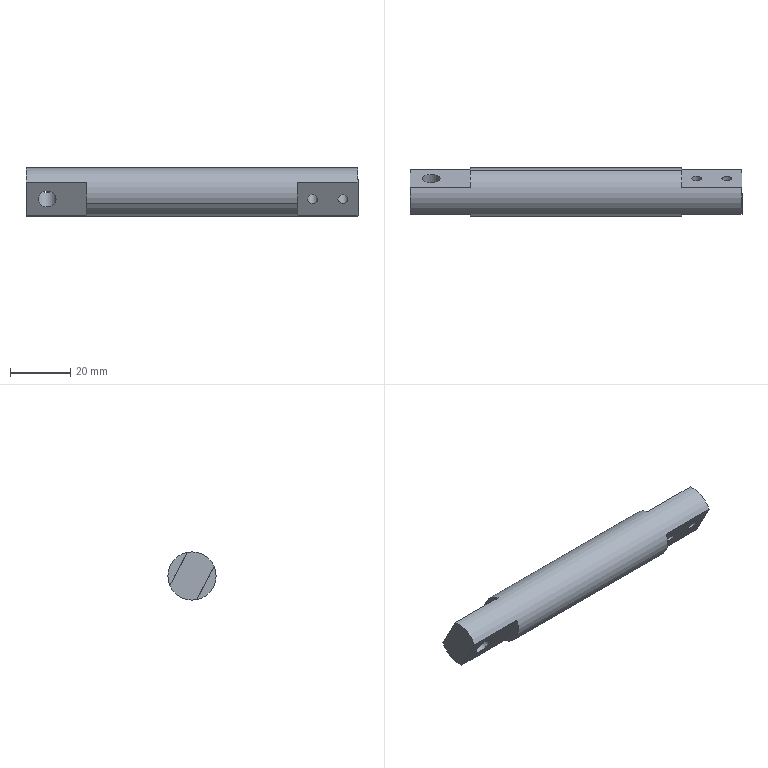Component | SolidWorks | BladeConnectingRod-1 | 1 solid | 18 faces | box 110 x 16 x 16 mm | volume 19575 mm3 | plane 10 | cylinder 8 | commonest cylinder face diameters 3.3 x4 6 x2 16 x2
build123d program:
from build123d import *

# Parameters (mm, degrees)
SKETCH1_R                    = 8
BOSS_EXTRUDE1_DEPTH          = 110
CUT_EXTRUDE1_DEPTH           = 20
F_6_0_6_DIAMETER_HOLE1_D     = 6
F_6_0_6_DIAMETER_HOLE1_DEPTH = 24
F_6_0_6_DIAMETER_HOLE1_TIP   = 1.803
CUT_EXTRUDE2_START           = -20
CUT_EXTRUDE2_DEPTH           = 20
M4_TAPPED_HOLE1_D            = 3.3
M4_TAPPED_HOLE1_DEPTH        = 13.5
M4_TAPPED_HOLE1_TIP          = 0.9914


with BuildPart() as part:
    # Sketch1 → Boss-Extrude1 (new body)
    with BuildSketch(Plane.XY):
        Circle(SKETCH1_R)
    extrude(amount=BOSS_EXTRUDE1_DEPTH)

    # Sketch2 → Cut-Extrude1 (cut)
    with BuildSketch(Plane(origin=(0, 0, 0), x_dir=(-1, 0, 0), z_dir=(0, 0, -1))):
        with BuildLine():
            Line((5, 6.245), (5, -6.245))
            ThreePointArc((5, -6.245), (8, 0), (5, 6.245))
        make_face()
        with BuildLine():
            Line((-5, 6.245), (-5, -6.245))
            ThreePointArc((-5, -6.245), (-8, 0), (-5, 6.245))
        make_face()
    extrude(amount=-CUT_EXTRUDE1_DEPTH, mode=Mode.SUBTRACT)

    # 6.0 _6_ Diameter Hole1
    with Locations(Plane(origin=(5, 0, 0), x_dir=(0, 0, -1), z_dir=(1, 0, 0))):
        with Locations((-7, 0)):
            Hole(F_6_0_6_DIAMETER_HOLE1_D / 2, depth=F_6_0_6_DIAMETER_HOLE1_DEPTH)
            with Locations((0, 0, -(F_6_0_6_DIAMETER_HOLE1_DEPTH + F_6_0_6_DIAMETER_HOLE1_TIP / 2))):  # 118° drill point
                Cone(0, F_6_0_6_DIAMETER_HOLE1_D / 2, F_6_0_6_DIAMETER_HOLE1_TIP, mode=Mode.SUBTRACT)

    # Sketch5 → Cut-Extrude2 (cut)
    with BuildSketch(Plane.XY.offset(110).offset(CUT_EXTRUDE2_START)):
        with BuildLine():
            Line((-5, 6.245), (-5, -6.245))
            ThreePointArc((-5, -6.245), (-8, 0), (-5, 6.245))
        make_face()
        with BuildLine():
            Line((5, 6.245), (5, -6.245))
            ThreePointArc((5, -6.245), (8, 0), (5, 6.245))
        make_face()
    extrude(amount=CUT_EXTRUDE2_DEPTH, mode=Mode.SUBTRACT)

    # M4 Tapped Hole1
    with Locations(Plane(origin=(5, 0, 0), x_dir=(0, 0, -1), z_dir=(1, 0, 0))):
        with Locations((-105, 0), (-95, 0)):
            Hole(M4_TAPPED_HOLE1_D / 2, depth=M4_TAPPED_HOLE1_DEPTH)
            with Locations((0, 0, -(M4_TAPPED_HOLE1_DEPTH + M4_TAPPED_HOLE1_TIP / 2))):  # 118° drill point
                Cone(0, M4_TAPPED_HOLE1_D / 2, M4_TAPPED_HOLE1_TIP, mode=Mode.SUBTRACT)


solid = part.part

# Placed as in the assembly
solid = solid.moved(Location((-280.317, -22.413, 172.524), (117.698, 90, 0)))
STEP:
#1=CARTESIAN_POINT('',(-6.837,-0.7081,6.884));
#2=VERTEX_POINT('',#1);
#3=CARTESIAN_POINT('',(-6.967,-0.7081,6.884));
#4=VERTEX_POINT('',#3);
#5=CARTESIAN_POINT('',(-6.902,-0.7081,6.884));
#6=DIRECTION('',(0.,-0.8854,-0.4648));
#7=DIRECTION('',(-1.,-0.,0.));
#8=AXIS2_PLACEMENT_3D('',#5,#6,#7);
#9=CIRCLE('',#8,0.06496);
#10=EDGE_CURVE('',#2,#4,#9,.T.);
#11=ORIENTED_EDGE('',*,*,#10,.F.);
#12=CARTESIAN_POINT('',(-6.837,-1.057,6.701));
#13=VERTEX_POINT('',#12);
#14=CARTESIAN_POINT('',(-6.837,-1.057,6.701));
#15=DIRECTION('',(0.,-0.8854,-0.4648));
#16=VECTOR('',#15,39.37);
#17=LINE('',#14,#16);
#18=EDGE_CURVE('',#2,#13,#17,.T.);
#19=ORIENTED_EDGE('',*,*,#18,.T.);
#20=CARTESIAN_POINT('',(-6.967,-1.057,6.701));
#21=VERTEX_POINT('',#20);
#22=CARTESIAN_POINT('',(-6.902,-1.057,6.701));
#23=DIRECTION('',(0.,-0.8854,-0.4648));
#24=DIRECTION('',(-1.,-0.,0.));
#25=AXIS2_PLACEMENT_3D('',#22,#23,#24);
#26=CIRCLE('',#25,0.06496);
#27=EDGE_CURVE('',#13,#21,#26,.T.);
#28=ORIENTED_EDGE('',*,*,#27,.T.);
#29=CARTESIAN_POINT('',(-6.967,-1.057,6.701));
#30=DIRECTION('',(0.,-0.8854,-0.4648));
#31=VECTOR('',#30,39.37);
#32=LINE('',#29,#31);
#33=EDGE_CURVE('',#4,#21,#32,.T.);
#34=ORIENTED_EDGE('',*,*,#33,.F.);
#35=EDGE_LOOP('',(#11,#19,#28,#34));
#36=FACE_OUTER_BOUND('',#35,.T.);
#37=CARTESIAN_POINT('',(-6.902,-1.057,6.701));
#38=DIRECTION('',(0.,-0.8854,-0.4648));
#39=DIRECTION('',(-1.,-0.,0.));
#40=AXIS2_PLACEMENT_3D('',#37,#38,#39);
#41=CYLINDRICAL_SURFACE('',#40,0.06496);
#42=ADVANCED_FACE('',(#36),#41,.F.);
#43=CARTESIAN_POINT('',(-7.231,-0.7081,6.884));
#44=VERTEX_POINT('',#43);
#45=CARTESIAN_POINT('',(-7.361,-0.7081,6.884));
#46=VERTEX_POINT('',#45);
#47=CARTESIAN_POINT('',(-7.296,-0.7081,6.884));
#48=DIRECTION('',(0.,-0.8854,-0.4648));
#49=DIRECTION('',(-1.,-0.,0.));
#50=AXIS2_PLACEMENT_3D('',#47,#48,#49);
#51=CIRCLE('',#50,0.06496);
#52=EDGE_CURVE('',#44,#46,#51,.T.);
#53=ORIENTED_EDGE('',*,*,#52,.F.);
#54=CARTESIAN_POINT('',(-7.231,-1.057,6.701));
#55=VERTEX_POINT('',#54);
#56=CARTESIAN_POINT('',(-7.231,-1.057,6.701));
#57=DIRECTION('',(0.,-0.8854,-0.4648));
#58=VECTOR('',#57,39.37);
#59=LINE('',#56,#58);
#60=EDGE_CURVE('',#44,#55,#59,.T.);
#61=ORIENTED_EDGE('',*,*,#60,.T.);
#62=CARTESIAN_POINT('',(-7.361,-1.057,6.701));
#63=VERTEX_POINT('',#62);
#64=CARTESIAN_POINT('',(-7.296,-1.057,6.701));
#65=DIRECTION('',(0.,-0.8854,-0.4648));
#66=DIRECTION('',(-1.,-0.,0.));
#67=AXIS2_PLACEMENT_3D('',#64,#65,#66);
#68=CIRCLE('',#67,0.06496);
#69=EDGE_CURVE('',#55,#63,#68,.T.);
#70=ORIENTED_EDGE('',*,*,#69,.T.);
#71=CARTESIAN_POINT('',(-7.361,-1.057,6.701));
#72=DIRECTION('',(0.,-0.8854,-0.4648));
#73=VECTOR('',#72,39.37);
#74=LINE('',#71,#73);
#75=EDGE_CURVE('',#46,#63,#74,.T.);
#76=ORIENTED_EDGE('',*,*,#75,.F.);
#77=EDGE_LOOP('',(#53,#61,#70,#76));
#78=FACE_OUTER_BOUND('',#77,.T.);
#79=CARTESIAN_POINT('',(-7.296,-1.057,6.701));
#80=DIRECTION('',(0.,-0.8854,-0.4648));
#81=DIRECTION('',(-1.,-0.,0.));
#82=AXIS2_PLACEMENT_3D('',#79,#80,#81);
#83=CYLINDRICAL_SURFACE('',#82,0.06496);
#84=ADVANCED_FACE('',(#78),#83,.F.);
#85=CARTESIAN_POINT('',(-10.642,-0.7081,6.884));
#86=VERTEX_POINT('',#85);
#87=CARTESIAN_POINT('',(-10.879,-0.7081,6.884));
#88=VERTEX_POINT('',#87);
#89=CARTESIAN_POINT('',(-10.76,-0.7081,6.884));
#90=DIRECTION('',(0.,-0.8854,-0.4648));
#91=DIRECTION('',(-1.,-0.,0.));
#92=AXIS2_PLACEMENT_3D('',#89,#90,#91);
#93=CIRCLE('',#92,0.1181);
#94=EDGE_CURVE('',#86,#88,#93,.T.);
#95=ORIENTED_EDGE('',*,*,#94,.F.);
#96=CARTESIAN_POINT('',(-10.642,-1.057,6.701));
#97=VERTEX_POINT('',#96);
#98=CARTESIAN_POINT('',(-10.642,-1.057,6.701));
#99=DIRECTION('',(0.,-0.8854,-0.4648));
#100=VECTOR('',#99,39.37);
#101=LINE('',#98,#100);
#102=EDGE_CURVE('',#86,#97,#101,.T.);
#103=ORIENTED_EDGE('',*,*,#102,.T.);
#104=CARTESIAN_POINT('',(-10.879,-1.057,6.701));
#105=VERTEX_POINT('',#104);
#106=CARTESIAN_POINT('',(-10.76,-1.057,6.701));
#107=DIRECTION('',(0.,-0.8854,-0.4648));
#108=DIRECTION('',(-1.,-0.,0.));
#109=AXIS2_PLACEMENT_3D('',#106,#107,#108);
#110=CIRCLE('',#109,0.1181);
#111=EDGE_CURVE('',#97,#105,#110,.T.);
#112=ORIENTED_EDGE('',*,*,#111,.T.);
#113=CARTESIAN_POINT('',(-10.879,-1.057,6.701));
#114=DIRECTION('',(0.,-0.8854,-0.4648));
#115=VECTOR('',#114,39.37);
#116=LINE('',#113,#115);
#117=EDGE_CURVE('',#88,#105,#116,.T.);
#118=ORIENTED_EDGE('',*,*,#117,.F.);
#119=EDGE_LOOP('',(#95,#103,#112,#118));
#120=FACE_OUTER_BOUND('',#119,.T.);
#121=CARTESIAN_POINT('',(-10.76,-1.057,6.701));
#122=DIRECTION('',(0.,-0.8854,-0.4648));
#123=DIRECTION('',(-1.,-0.,0.));
#124=AXIS2_PLACEMENT_3D('',#121,#122,#123);
#125=CYLINDRICAL_SURFACE('',#124,0.1181);
#126=ADVANCED_FACE('',(#120),#125,.F.);
#127=CARTESIAN_POINT('',(-7.493,-1.161,6.646));
#128=VERTEX_POINT('',#127);
#129=CARTESIAN_POINT('',(-7.493,-0.9424,6.483));
#130=VERTEX_POINT('',#129);
#131=CARTESIAN_POINT('',(-7.493,-0.8824,6.792));
#132=DIRECTION('',(1.,0.,0.));
#133=DIRECTION('',(0.,-0.8854,-0.4648));
#134=AXIS2_PLACEMENT_3D('',#131,#132,#133);
#135=CIRCLE('',#134,0.315);
#136=EDGE_CURVE('',#128,#130,#135,.T.);
#137=ORIENTED_EDGE('',*,*,#136,.F.);
#138=CARTESIAN_POINT('',(-10.249,-1.161,6.646));
#139=VERTEX_POINT('',#138);
#140=CARTESIAN_POINT('',(-6.705,-1.161,6.646));
#141=DIRECTION('',(-1.,-0.,-0.));
#142=VECTOR('',#141,39.37);
#143=LINE('',#140,#142);
#144=EDGE_CURVE('',#128,#139,#143,.T.);
#145=ORIENTED_EDGE('',*,*,#144,.T.);
#146=CARTESIAN_POINT('',(-10.249,-0.9424,6.483));
#147=VERTEX_POINT('',#146);
#148=CARTESIAN_POINT('',(-10.249,-0.8824,6.792));
#149=DIRECTION('',(-1.,-0.,-0.));
#150=DIRECTION('',(0.,0.8854,0.4648));
#151=AXIS2_PLACEMENT_3D('',#148,#149,#150);
#152=CIRCLE('',#151,0.315);
#153=EDGE_CURVE('',#147,#139,#152,.T.);
#154=ORIENTED_EDGE('',*,*,#153,.F.);
#155=CARTESIAN_POINT('',(-11.036,-0.9424,6.483));
#156=VERTEX_POINT('',#155);
#157=CARTESIAN_POINT('',(-10.249,-0.9424,6.483));
#158=DIRECTION('',(-1.,-0.,-0.));
#159=VECTOR('',#158,39.37);
#160=LINE('',#157,#159);
#161=EDGE_CURVE('',#147,#156,#160,.T.);
#162=ORIENTED_EDGE('',*,*,#161,.T.);
#163=CARTESIAN_POINT('',(-11.036,-0.5938,6.666));
#164=VERTEX_POINT('',#163);
#165=CARTESIAN_POINT('',(-11.036,-0.8824,6.792));
#166=DIRECTION('',(1.,0.,0.));
#167=DIRECTION('',(0.,-0.8854,-0.4648));
#168=AXIS2_PLACEMENT_3D('',#165,#166,#167);
#169=CIRCLE('',#168,0.315);
#170=EDGE_CURVE('',#156,#164,#169,.T.);
#171=ORIENTED_EDGE('',*,*,#170,.T.);
#172=CARTESIAN_POINT('',(-10.249,-0.5938,6.666));
#173=VERTEX_POINT('',#172);
#174=CARTESIAN_POINT('',(-10.249,-0.5938,6.666));
#175=DIRECTION('',(-1.,-0.,-0.));
#176=VECTOR('',#175,39.37);
#177=LINE('',#174,#176);
#178=EDGE_CURVE('',#173,#164,#177,.T.);
#179=ORIENTED_EDGE('',*,*,#178,.F.);
#180=CARTESIAN_POINT('',(-10.249,-0.6035,6.939));
#181=VERTEX_POINT('',#180);
#182=CARTESIAN_POINT('',(-10.249,-0.8824,6.792));
#183=DIRECTION('',(-1.,-0.,-0.));
#184=DIRECTION('',(0.,0.8854,0.4648));
#185=AXIS2_PLACEMENT_3D('',#182,#183,#184);
#186=CIRCLE('',#185,0.315);
#187=EDGE_CURVE('',#181,#173,#186,.T.);
#188=ORIENTED_EDGE('',*,*,#187,.F.);
#189=CARTESIAN_POINT('',(-7.493,-0.6035,6.939));
#190=VERTEX_POINT('',#189);
#191=CARTESIAN_POINT('',(-6.705,-0.6035,6.939));
#192=DIRECTION('',(-1.,-0.,-0.));
#193=VECTOR('',#192,39.37);
#194=LINE('',#191,#193);
#195=EDGE_CURVE('',#190,#181,#194,.T.);
#196=ORIENTED_EDGE('',*,*,#195,.F.);
#197=CARTESIAN_POINT('',(-7.493,-0.5938,6.666));
#198=VERTEX_POINT('',#197);
#199=CARTESIAN_POINT('',(-7.493,-0.8824,6.792));
#200=DIRECTION('',(1.,0.,0.));
#201=DIRECTION('',(0.,-0.8854,-0.4648));
#202=AXIS2_PLACEMENT_3D('',#199,#200,#201);
#203=CIRCLE('',#202,0.315);
#204=EDGE_CURVE('',#198,#190,#203,.T.);
#205=ORIENTED_EDGE('',*,*,#204,.F.);
#206=CARTESIAN_POINT('',(-6.705,-0.5938,6.666));
#207=VERTEX_POINT('',#206);
#208=CARTESIAN_POINT('',(-7.493,-0.5938,6.666));
#209=DIRECTION('',(1.,0.,0.));
#210=VECTOR('',#209,39.37);
#211=LINE('',#208,#210);
#212=EDGE_CURVE('',#198,#207,#211,.T.);
#213=ORIENTED_EDGE('',*,*,#212,.T.);
#214=CARTESIAN_POINT('',(-6.705,-0.9424,6.483));
#215=VERTEX_POINT('',#214);
#216=CARTESIAN_POINT('',(-6.705,-0.8824,6.792));
#217=DIRECTION('',(1.,0.,0.));
#218=DIRECTION('',(0.,-0.8854,-0.4648));
#219=AXIS2_PLACEMENT_3D('',#216,#217,#218);
#220=CIRCLE('',#219,0.315);
#221=EDGE_CURVE('',#215,#207,#220,.T.);
#222=ORIENTED_EDGE('',*,*,#221,.F.);
#223=CARTESIAN_POINT('',(-7.493,-0.9424,6.483));
#224=DIRECTION('',(1.,0.,0.));
#225=VECTOR('',#224,39.37);
#226=LINE('',#223,#225);
#227=EDGE_CURVE('',#130,#215,#226,.T.);
#228=ORIENTED_EDGE('',*,*,#227,.F.);
#229=EDGE_LOOP('',(#137,#145,#154,#162,#171,#179,#188,#196,#205,#213,#222,#228));
#230=FACE_OUTER_BOUND('',#229,.T.);
#231=CARTESIAN_POINT('',(-6.705,-0.8824,6.792));
#232=DIRECTION('',(-1.,-0.,-0.));
#233=DIRECTION('',(-0.,0.8854,0.4648));
#234=AXIS2_PLACEMENT_3D('',#231,#232,#233);
#235=CYLINDRICAL_SURFACE('',#234,0.315);
#236=ADVANCED_FACE('',(#230),#235,.T.);
#237=ORIENTED_EDGE('',*,*,#144,.F.);
#238=CARTESIAN_POINT('',(-7.493,-1.171,6.918));
#239=VERTEX_POINT('',#238);
#240=CARTESIAN_POINT('',(-7.493,-0.8824,6.792));
#241=DIRECTION('',(1.,0.,0.));
#242=DIRECTION('',(0.,-0.8854,-0.4648));
#243=AXIS2_PLACEMENT_3D('',#240,#241,#242);
#244=CIRCLE('',#243,0.315);
#245=EDGE_CURVE('',#239,#128,#244,.T.);
#246=ORIENTED_EDGE('',*,*,#245,.F.);
#247=CARTESIAN_POINT('',(-6.705,-1.171,6.918));
#248=VERTEX_POINT('',#247);
#249=CARTESIAN_POINT('',(-7.493,-1.171,6.918));
#250=DIRECTION('',(1.,0.,0.));
#251=VECTOR('',#250,39.37);
#252=LINE('',#249,#251);
#253=EDGE_CURVE('',#239,#248,#252,.T.);
#254=ORIENTED_EDGE('',*,*,#253,.T.);
#255=CARTESIAN_POINT('',(-6.705,-0.8224,7.101));
#256=VERTEX_POINT('',#255);
#257=CARTESIAN_POINT('',(-6.705,-0.8824,6.792));
#258=DIRECTION('',(1.,0.,0.));
#259=DIRECTION('',(0.,-0.8854,-0.4648));
#260=AXIS2_PLACEMENT_3D('',#257,#258,#259);
#261=CIRCLE('',#260,0.315);
#262=EDGE_CURVE('',#256,#248,#261,.T.);
#263=ORIENTED_EDGE('',*,*,#262,.F.);
#264=CARTESIAN_POINT('',(-7.493,-0.8224,7.101));
#265=VERTEX_POINT('',#264);
#266=CARTESIAN_POINT('',(-7.493,-0.8224,7.101));
#267=DIRECTION('',(1.,0.,0.));
#268=VECTOR('',#267,39.37);
#269=LINE('',#266,#268);
#270=EDGE_CURVE('',#265,#256,#269,.T.);
#271=ORIENTED_EDGE('',*,*,#270,.F.);
#272=CARTESIAN_POINT('',(-7.493,-0.8824,6.792));
#273=DIRECTION('',(1.,0.,0.));
#274=DIRECTION('',(0.,-0.8854,-0.4648));
#275=AXIS2_PLACEMENT_3D('',#272,#273,#274);
#276=CIRCLE('',#275,0.315);
#277=EDGE_CURVE('',#190,#265,#276,.T.);
#278=ORIENTED_EDGE('',*,*,#277,.F.);
#279=ORIENTED_EDGE('',*,*,#195,.T.);
#280=CARTESIAN_POINT('',(-10.249,-0.8224,7.101));
#281=VERTEX_POINT('',#280);
#282=CARTESIAN_POINT('',(-10.249,-0.8824,6.792));
#283=DIRECTION('',(-1.,-0.,-0.));
#284=DIRECTION('',(0.,0.8854,0.4648));
#285=AXIS2_PLACEMENT_3D('',#282,#283,#284);
#286=CIRCLE('',#285,0.315);
#287=EDGE_CURVE('',#281,#181,#286,.T.);
#288=ORIENTED_EDGE('',*,*,#287,.F.);
#289=CARTESIAN_POINT('',(-11.036,-0.8224,7.101));
#290=VERTEX_POINT('',#289);
#291=CARTESIAN_POINT('',(-10.249,-0.8224,7.101));
#292=DIRECTION('',(-1.,-0.,-0.));
#293=VECTOR('',#292,39.37);
#294=LINE('',#291,#293);
#295=EDGE_CURVE('',#281,#290,#294,.T.);
#296=ORIENTED_EDGE('',*,*,#295,.T.);
#297=CARTESIAN_POINT('',(-11.036,-1.171,6.918));
#298=VERTEX_POINT('',#297);
#299=CARTESIAN_POINT('',(-11.036,-0.8824,6.792));
#300=DIRECTION('',(1.,0.,0.));
#301=DIRECTION('',(0.,-0.8854,-0.4648));
#302=AXIS2_PLACEMENT_3D('',#299,#300,#301);
#303=CIRCLE('',#302,0.315);
#304=EDGE_CURVE('',#290,#298,#303,.T.);
#305=ORIENTED_EDGE('',*,*,#304,.T.);
#306=CARTESIAN_POINT('',(-10.249,-1.171,6.918));
#307=VERTEX_POINT('',#306);
#308=CARTESIAN_POINT('',(-10.249,-1.171,6.918));
#309=DIRECTION('',(-1.,-0.,-0.));
#310=VECTOR('',#309,39.37);
#311=LINE('',#308,#310);
#312=EDGE_CURVE('',#307,#298,#311,.T.);
#313=ORIENTED_EDGE('',*,*,#312,.F.);
#314=CARTESIAN_POINT('',(-10.249,-0.8824,6.792));
#315=DIRECTION('',(-1.,-0.,-0.));
#316=DIRECTION('',(0.,0.8854,0.4648));
#317=AXIS2_PLACEMENT_3D('',#314,#315,#316);
#318=CIRCLE('',#317,0.315);
#319=EDGE_CURVE('',#139,#307,#318,.T.);
#320=ORIENTED_EDGE('',*,*,#319,.F.);
#321=EDGE_LOOP('',(#237,#246,#254,#263,#271,#278,#279,#288,#296,#305,#313,#320));
#322=FACE_OUTER_BOUND('',#321,.T.);
#323=CARTESIAN_POINT('',(-6.705,-0.8824,6.792));
#324=DIRECTION('',(-1.,-0.,-0.));
#325=DIRECTION('',(-0.,0.8854,0.4648));
#326=AXIS2_PLACEMENT_3D('',#323,#324,#325);
#327=CYLINDRICAL_SURFACE('',#326,0.315);
#328=ADVANCED_FACE('',(#322),#327,.T.);
#329=CARTESIAN_POINT('',(-6.705,-0.5938,6.666));
#330=DIRECTION('',(-0.,0.4648,-0.8854));
#331=VECTOR('',#330,39.37);
#332=LINE('',#329,#331);
#333=EDGE_CURVE('',#256,#207,#332,.T.);
#334=ORIENTED_EDGE('',*,*,#333,.F.);
#335=ORIENTED_EDGE('',*,*,#262,.T.);
#336=CARTESIAN_POINT('',(-6.705,-0.9424,6.483));
#337=DIRECTION('',(0.,-0.4648,0.8854));
#338=VECTOR('',#337,39.37);
#339=LINE('',#336,#338);
#340=EDGE_CURVE('',#215,#248,#339,.T.);
#341=ORIENTED_EDGE('',*,*,#340,.F.);
#342=ORIENTED_EDGE('',*,*,#221,.T.);
#343=EDGE_LOOP('',(#334,#335,#341,#342));
#344=FACE_OUTER_BOUND('',#343,.T.);
#345=CARTESIAN_POINT('',(-6.705,-0.8824,6.792));
#346=DIRECTION('',(1.,0.,0.));
#347=DIRECTION('',(0.,-0.8854,-0.4648));
#348=AXIS2_PLACEMENT_3D('',#345,#346,#347);
#349=PLANE('',#348);
#350=ADVANCED_FACE('',(#344),#349,.T.);
#351=ORIENTED_EDGE('',*,*,#304,.F.);
#352=CARTESIAN_POINT('',(-11.036,-0.5938,6.666));
#353=DIRECTION('',(0.,-0.4648,0.8854));
#354=VECTOR('',#353,39.37);
#355=LINE('',#352,#354);
#356=EDGE_CURVE('',#164,#290,#355,.T.);
#357=ORIENTED_EDGE('',*,*,#356,.F.);
#358=ORIENTED_EDGE('',*,*,#170,.F.);
#359=CARTESIAN_POINT('',(-11.036,-0.9424,6.483));
#360=DIRECTION('',(-0.,0.4648,-0.8854));
#361=VECTOR('',#360,39.37);
#362=LINE('',#359,#361);
#363=EDGE_CURVE('',#298,#156,#362,.T.);
#364=ORIENTED_EDGE('',*,*,#363,.F.);
#365=EDGE_LOOP('',(#351,#357,#358,#364));
#366=FACE_OUTER_BOUND('',#365,.T.);
#367=CARTESIAN_POINT('',(-11.036,-0.8824,6.792));
#368=DIRECTION('',(1.,0.,0.));
#369=DIRECTION('',(0.,-0.8854,-0.4648));
#370=AXIS2_PLACEMENT_3D('',#367,#368,#369);
#371=PLANE('',#370);
#372=ADVANCED_FACE('',(#366),#371,.F.);
#373=CARTESIAN_POINT('',(-10.76,-1.057,6.701));
#374=DIRECTION('',(0.,-0.8854,-0.4648));
#375=DIRECTION('',(-1.,-0.,0.));
#376=AXIS2_PLACEMENT_3D('',#373,#374,#375);
#377=CIRCLE('',#376,0.1181);
#378=EDGE_CURVE('',#105,#97,#377,.T.);
#379=ORIENTED_EDGE('',*,*,#378,.F.);
#380=ORIENTED_EDGE('',*,*,#111,.F.);
#381=EDGE_LOOP('',(#379,#380));
#382=FACE_BOUND('',#381,.T.);
#383=ORIENTED_EDGE('',*,*,#363,.T.);
#384=ORIENTED_EDGE('',*,*,#161,.F.);
#385=CARTESIAN_POINT('',(-10.249,-0.9424,6.483));
#386=DIRECTION('',(-0.,0.4648,-0.8854));
#387=VECTOR('',#386,39.37);
#388=LINE('',#385,#387);
#389=EDGE_CURVE('',#307,#147,#388,.T.);
#390=ORIENTED_EDGE('',*,*,#389,.F.);
#391=ORIENTED_EDGE('',*,*,#312,.T.);
#392=EDGE_LOOP('',(#383,#384,#390,#391));
#393=FACE_OUTER_BOUND('',#392,.T.);
#394=CARTESIAN_POINT('',(-10.249,-0.9424,6.483));
#395=DIRECTION('',(-0.,0.8854,0.4648));
#396=DIRECTION('',(1.,0.,0.));
#397=AXIS2_PLACEMENT_3D('',#394,#395,#396);
#398=PLANE('',#397);
#399=ADVANCED_FACE('',(#382,#393),#398,.F.);
#400=ORIENTED_EDGE('',*,*,#153,.T.);
#401=ORIENTED_EDGE('',*,*,#319,.T.);
#402=ORIENTED_EDGE('',*,*,#389,.T.);
#403=EDGE_LOOP('',(#400,#401,#402));
#404=FACE_OUTER_BOUND('',#403,.T.);
#405=CARTESIAN_POINT('',(-10.249,-0.8824,6.792));
#406=DIRECTION('',(-1.,-0.,-0.));
#407=DIRECTION('',(-0.,0.8854,0.4648));
#408=AXIS2_PLACEMENT_3D('',#405,#406,#407);
#409=PLANE('',#408);
#410=ADVANCED_FACE('',(#404),#409,.T.);
#411=CARTESIAN_POINT('',(-10.76,-0.7081,6.884));
#412=DIRECTION('',(0.,-0.8854,-0.4648));
#413=DIRECTION('',(-1.,-0.,0.));
#414=AXIS2_PLACEMENT_3D('',#411,#412,#413);
#415=CIRCLE('',#414,0.1181);
#416=EDGE_CURVE('',#88,#86,#415,.T.);
#417=ORIENTED_EDGE('',*,*,#416,.T.);
#418=ORIENTED_EDGE('',*,*,#94,.T.);
#419=EDGE_LOOP('',(#417,#418));
#420=FACE_BOUND('',#419,.T.);
#421=ORIENTED_EDGE('',*,*,#356,.T.);
#422=ORIENTED_EDGE('',*,*,#295,.F.);
#423=CARTESIAN_POINT('',(-10.249,-0.5938,6.666));
#424=DIRECTION('',(0.,-0.4648,0.8854));
#425=VECTOR('',#424,39.37);
#426=LINE('',#423,#425);
#427=EDGE_CURVE('',#173,#281,#426,.T.);
#428=ORIENTED_EDGE('',*,*,#427,.F.);
#429=ORIENTED_EDGE('',*,*,#178,.T.);
#430=EDGE_LOOP('',(#421,#422,#428,#429));
#431=FACE_OUTER_BOUND('',#430,.T.);
#432=CARTESIAN_POINT('',(-10.249,-0.5938,6.666));
#433=DIRECTION('',(0.,-0.8854,-0.4648));
#434=DIRECTION('',(-1.,-0.,-0.));
#435=AXIS2_PLACEMENT_3D('',#432,#433,#434);
#436=PLANE('',#435);
#437=ADVANCED_FACE('',(#420,#431),#436,.F.);
#438=ORIENTED_EDGE('',*,*,#287,.T.);
#439=ORIENTED_EDGE('',*,*,#187,.T.);
#440=ORIENTED_EDGE('',*,*,#427,.T.);
#441=EDGE_LOOP('',(#438,#439,#440));
#442=FACE_OUTER_BOUND('',#441,.T.);
#443=CARTESIAN_POINT('',(-10.249,-0.8824,6.792));
#444=DIRECTION('',(-1.,-0.,-0.));
#445=DIRECTION('',(-0.,0.8854,0.4648));
#446=AXIS2_PLACEMENT_3D('',#443,#444,#445);
#447=PLANE('',#446);
#448=ADVANCED_FACE('',(#442),#447,.T.);
#449=ORIENTED_EDGE('',*,*,#102,.F.);
#450=ORIENTED_EDGE('',*,*,#416,.F.);
#451=ORIENTED_EDGE('',*,*,#117,.T.);
#452=ORIENTED_EDGE('',*,*,#378,.T.);
#453=EDGE_LOOP('',(#449,#450,#451,#452));
#454=FACE_OUTER_BOUND('',#453,.T.);
#455=CARTESIAN_POINT('',(-10.76,-1.057,6.701));
#456=DIRECTION('',(0.,-0.8854,-0.4648));
#457=DIRECTION('',(-1.,-0.,0.));
#458=AXIS2_PLACEMENT_3D('',#455,#456,#457);
#459=CYLINDRICAL_SURFACE('',#458,0.1181);
#460=ADVANCED_FACE('',(#454),#459,.F.);
#461=CARTESIAN_POINT('',(-6.902,-1.057,6.701));
#462=DIRECTION('',(0.,-0.8854,-0.4648));
#463=DIRECTION('',(-1.,-0.,0.));
#464=AXIS2_PLACEMENT_3D('',#461,#462,#463);
#465=CIRCLE('',#464,0.06496);
#466=EDGE_CURVE('',#21,#13,#465,.T.);
#467=ORIENTED_EDGE('',*,*,#466,.F.);
#468=ORIENTED_EDGE('',*,*,#27,.F.);
#469=EDGE_LOOP('',(#467,#468));
#470=FACE_BOUND('',#469,.T.);
#471=CARTESIAN_POINT('',(-7.296,-1.057,6.701));
#472=DIRECTION('',(0.,-0.8854,-0.4648));
#473=DIRECTION('',(-1.,-0.,0.));
#474=AXIS2_PLACEMENT_3D('',#471,#472,#473);
#475=CIRCLE('',#474,0.06496);
#476=EDGE_CURVE('',#63,#55,#475,.T.);
#477=ORIENTED_EDGE('',*,*,#476,.F.);
#478=ORIENTED_EDGE('',*,*,#69,.F.);
#479=EDGE_LOOP('',(#477,#478));
#480=FACE_BOUND('',#479,.T.);
#481=ORIENTED_EDGE('',*,*,#340,.T.);
#482=ORIENTED_EDGE('',*,*,#253,.F.);
#483=CARTESIAN_POINT('',(-7.493,-0.9424,6.483));
#484=DIRECTION('',(0.,-0.4648,0.8854));
#485=VECTOR('',#484,39.37);
#486=LINE('',#483,#485);
#487=EDGE_CURVE('',#130,#239,#486,.T.);
#488=ORIENTED_EDGE('',*,*,#487,.F.);
#489=ORIENTED_EDGE('',*,*,#227,.T.);
#490=EDGE_LOOP('',(#481,#482,#488,#489));
#491=FACE_OUTER_BOUND('',#490,.T.);
#492=CARTESIAN_POINT('',(-7.493,-0.9424,6.483));
#493=DIRECTION('',(-0.,0.8854,0.4648));
#494=DIRECTION('',(1.,0.,0.));
#495=AXIS2_PLACEMENT_3D('',#492,#493,#494);
#496=PLANE('',#495);
#497=ADVANCED_FACE('',(#470,#480,#491),#496,.F.);
#498=ORIENTED_EDGE('',*,*,#245,.T.);
#499=ORIENTED_EDGE('',*,*,#136,.T.);
#500=ORIENTED_EDGE('',*,*,#487,.T.);
#501=EDGE_LOOP('',(#498,#499,#500));
#502=FACE_OUTER_BOUND('',#501,.T.);
#503=CARTESIAN_POINT('',(-7.493,-0.8824,6.792));
#504=DIRECTION('',(1.,0.,0.));
#505=DIRECTION('',(0.,-0.8854,-0.4648));
#506=AXIS2_PLACEMENT_3D('',#503,#504,#505);
#507=PLANE('',#506);
#508=ADVANCED_FACE('',(#502),#507,.T.);
#509=CARTESIAN_POINT('',(-6.902,-0.7081,6.884));
#510=DIRECTION('',(0.,-0.8854,-0.4648));
#511=DIRECTION('',(-1.,-0.,0.));
#512=AXIS2_PLACEMENT_3D('',#509,#510,#511);
#513=CIRCLE('',#512,0.06496);
#514=EDGE_CURVE('',#4,#2,#513,.T.);
#515=ORIENTED_EDGE('',*,*,#514,.T.);
#516=ORIENTED_EDGE('',*,*,#10,.T.);
#517=EDGE_LOOP('',(#515,#516));
#518=FACE_BOUND('',#517,.T.);
#519=CARTESIAN_POINT('',(-7.296,-0.7081,6.884));
#520=DIRECTION('',(0.,-0.8854,-0.4648));
#521=DIRECTION('',(-1.,-0.,0.));
#522=AXIS2_PLACEMENT_3D('',#519,#520,#521);
#523=CIRCLE('',#522,0.06496);
#524=EDGE_CURVE('',#46,#44,#523,.T.);
#525=ORIENTED_EDGE('',*,*,#524,.T.);
#526=ORIENTED_EDGE('',*,*,#52,.T.);
#527=EDGE_LOOP('',(#525,#526));
#528=FACE_BOUND('',#527,.T.);
#529=ORIENTED_EDGE('',*,*,#333,.T.);
#530=ORIENTED_EDGE('',*,*,#212,.F.);
#531=CARTESIAN_POINT('',(-7.493,-0.5938,6.666));
#532=DIRECTION('',(-0.,0.4648,-0.8854));
#533=VECTOR('',#532,39.37);
#534=LINE('',#531,#533);
#535=EDGE_CURVE('',#265,#198,#534,.T.);
#536=ORIENTED_EDGE('',*,*,#535,.F.);
#537=ORIENTED_EDGE('',*,*,#270,.T.);
#538=EDGE_LOOP('',(#529,#530,#536,#537));
#539=FACE_OUTER_BOUND('',#538,.T.);
#540=CARTESIAN_POINT('',(-7.493,-0.5938,6.666));
#541=DIRECTION('',(0.,-0.8854,-0.4648));
#542=DIRECTION('',(-1.,-0.,-0.));
#543=AXIS2_PLACEMENT_3D('',#540,#541,#542);
#544=PLANE('',#543);
#545=ADVANCED_FACE('',(#518,#528,#539),#544,.F.);
#546=ORIENTED_EDGE('',*,*,#204,.T.);
#547=ORIENTED_EDGE('',*,*,#277,.T.);
#548=ORIENTED_EDGE('',*,*,#535,.T.);
#549=EDGE_LOOP('',(#546,#547,#548));
#550=FACE_OUTER_BOUND('',#549,.T.);
#551=CARTESIAN_POINT('',(-7.493,-0.8824,6.792));
#552=DIRECTION('',(1.,0.,0.));
#553=DIRECTION('',(0.,-0.8854,-0.4648));
#554=AXIS2_PLACEMENT_3D('',#551,#552,#553);
#555=PLANE('',#554);
#556=ADVANCED_FACE('',(#550),#555,.T.);
#557=ORIENTED_EDGE('',*,*,#60,.F.);
#558=ORIENTED_EDGE('',*,*,#524,.F.);
#559=ORIENTED_EDGE('',*,*,#75,.T.);
#560=ORIENTED_EDGE('',*,*,#476,.T.);
#561=EDGE_LOOP('',(#557,#558,#559,#560));
#562=FACE_OUTER_BOUND('',#561,.T.);
#563=CARTESIAN_POINT('',(-7.296,-1.057,6.701));
#564=DIRECTION('',(0.,-0.8854,-0.4648));
#565=DIRECTION('',(-1.,-0.,0.));
#566=AXIS2_PLACEMENT_3D('',#563,#564,#565);
#567=CYLINDRICAL_SURFACE('',#566,0.06496);
#568=ADVANCED_FACE('',(#562),#567,.F.);
#569=ORIENTED_EDGE('',*,*,#18,.F.);
#570=ORIENTED_EDGE('',*,*,#514,.F.);
#571=ORIENTED_EDGE('',*,*,#33,.T.);
#572=ORIENTED_EDGE('',*,*,#466,.T.);
#573=EDGE_LOOP('',(#569,#570,#571,#572));
#574=FACE_OUTER_BOUND('',#573,.T.);
#575=CARTESIAN_POINT('',(-6.902,-1.057,6.701));
#576=DIRECTION('',(0.,-0.8854,-0.4648));
#577=DIRECTION('',(-1.,-0.,0.));
#578=AXIS2_PLACEMENT_3D('',#575,#576,#577);
#579=CYLINDRICAL_SURFACE('',#578,0.06496);
#580=ADVANCED_FACE('',(#574),#579,.F.);
#581=CLOSED_SHELL('',(#42,#84,#126,#236,#328,#350,#372,#399,#410,#437,#448,#460,#497,#508,#545,#556,#568,#580));
#582=MANIFOLD_SOLID_BREP('',#581);
#583=CARTESIAN_POINT('',(0.,0.,0.));
#584=DIRECTION('',(0.,0.,1.));
#585=DIRECTION('',(1.,0.,0.));
#586=AXIS2_PLACEMENT_3D('',#583,#584,#585);
#587=(LENGTH_UNIT()NAMED_UNIT(*)SI_UNIT($,.METRE.));
#588=LENGTH_MEASURE_WITH_UNIT(LENGTH_MEASURE(0.0254),#587);
#589=DIMENSIONAL_EXPONENTS(1.,0.,0.,0.,0.,0.,0.);
#590=(CONVERSION_BASED_UNIT('',#588)LENGTH_UNIT()NAMED_UNIT(#589));
#591=UNCERTAINTY_MEASURE_WITH_UNIT(LENGTH_MEASURE(0.00001),#590,'','');
#592=(NAMED_UNIT(*)PLANE_ANGLE_UNIT()SI_UNIT($,.RADIAN.));
#593=(NAMED_UNIT(*)SI_UNIT($,.STERADIAN.)SOLID_ANGLE_UNIT());
#594=(GEOMETRIC_REPRESENTATION_CONTEXT(3)GLOBAL_UNCERTAINTY_ASSIGNED_CONTEXT((#591))GLOBAL_UNIT_ASSIGNED_CONTEXT((#590,#592,#593))REPRESENTATION_CONTEXT('',''));
#595=ADVANCED_BREP_SHAPE_REPRESENTATION('',(#582,#586),#594);
#596=COLOUR_RGB('',0.7922,0.8196,0.9333);
#597=FILL_AREA_STYLE_COLOUR('',#596);
#598=FILL_AREA_STYLE('',(#597));
#599=SURFACE_STYLE_FILL_AREA(#598);
#600=SURFACE_SIDE_STYLE('',(#599));
#601=SURFACE_STYLE_USAGE(.BOTH.,#600);
#602=PRESENTATION_STYLE_ASSIGNMENT((#601));
#603=STYLED_ITEM('',(#602),#582);
#604=PRESENTATION_LAYER_ASSIGNMENT('','',(#603));
#605=(LENGTH_UNIT()NAMED_UNIT(*)SI_UNIT($,.METRE.));
#606=LENGTH_MEASURE_WITH_UNIT(LENGTH_MEASURE(0.0254),#605);
#607=DIMENSIONAL_EXPONENTS(1.,0.,0.,0.,0.,0.,0.);
#608=(CONVERSION_BASED_UNIT('',#606)LENGTH_UNIT()NAMED_UNIT(#607));
#609=UNCERTAINTY_MEASURE_WITH_UNIT(LENGTH_MEASURE(0.00001),#608,'','');
#610=(NAMED_UNIT(*)PLANE_ANGLE_UNIT()SI_UNIT($,.RADIAN.));
#611=(NAMED_UNIT(*)SI_UNIT($,.STERADIAN.)SOLID_ANGLE_UNIT());
#612=(GEOMETRIC_REPRESENTATION_CONTEXT(3)GLOBAL_UNCERTAINTY_ASSIGNED_CONTEXT((#609))GLOBAL_UNIT_ASSIGNED_CONTEXT((#608,#610,#611))REPRESENTATION_CONTEXT('',''));
#613=MECHANICAL_DESIGN_GEOMETRIC_PRESENTATION_REPRESENTATION('',(#603),#612);